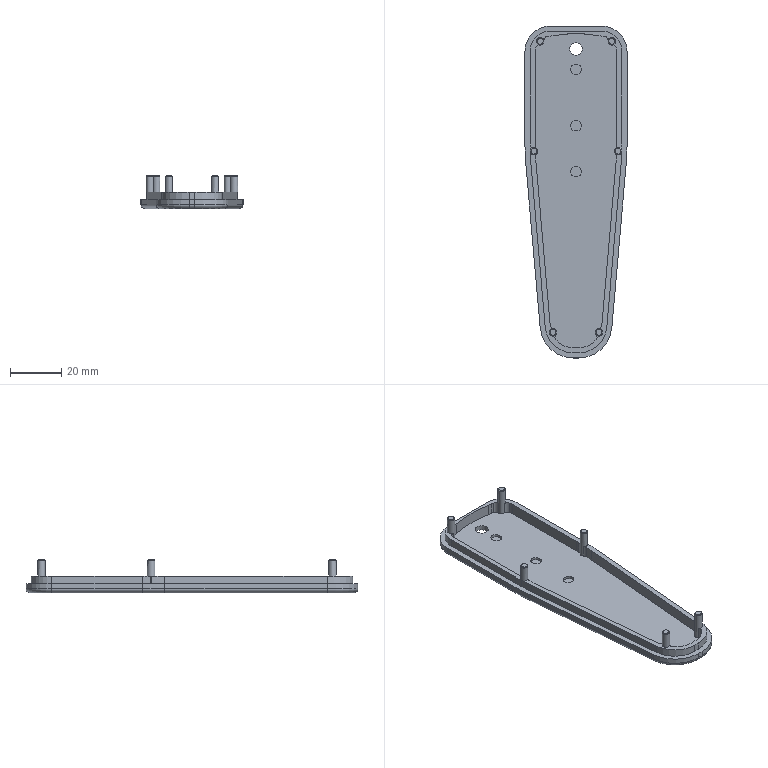Component | NX | CASING_2 | 1 solid | 98 faces | volume 12673 mm3 | cylinder 55 | plane 31 | torus 6 | cone 6 | commonest cylinder face diameters 3 x18 2.9 x6 196 x4 192 x4 12 x4 4.2 x3 18 x2 22 x2